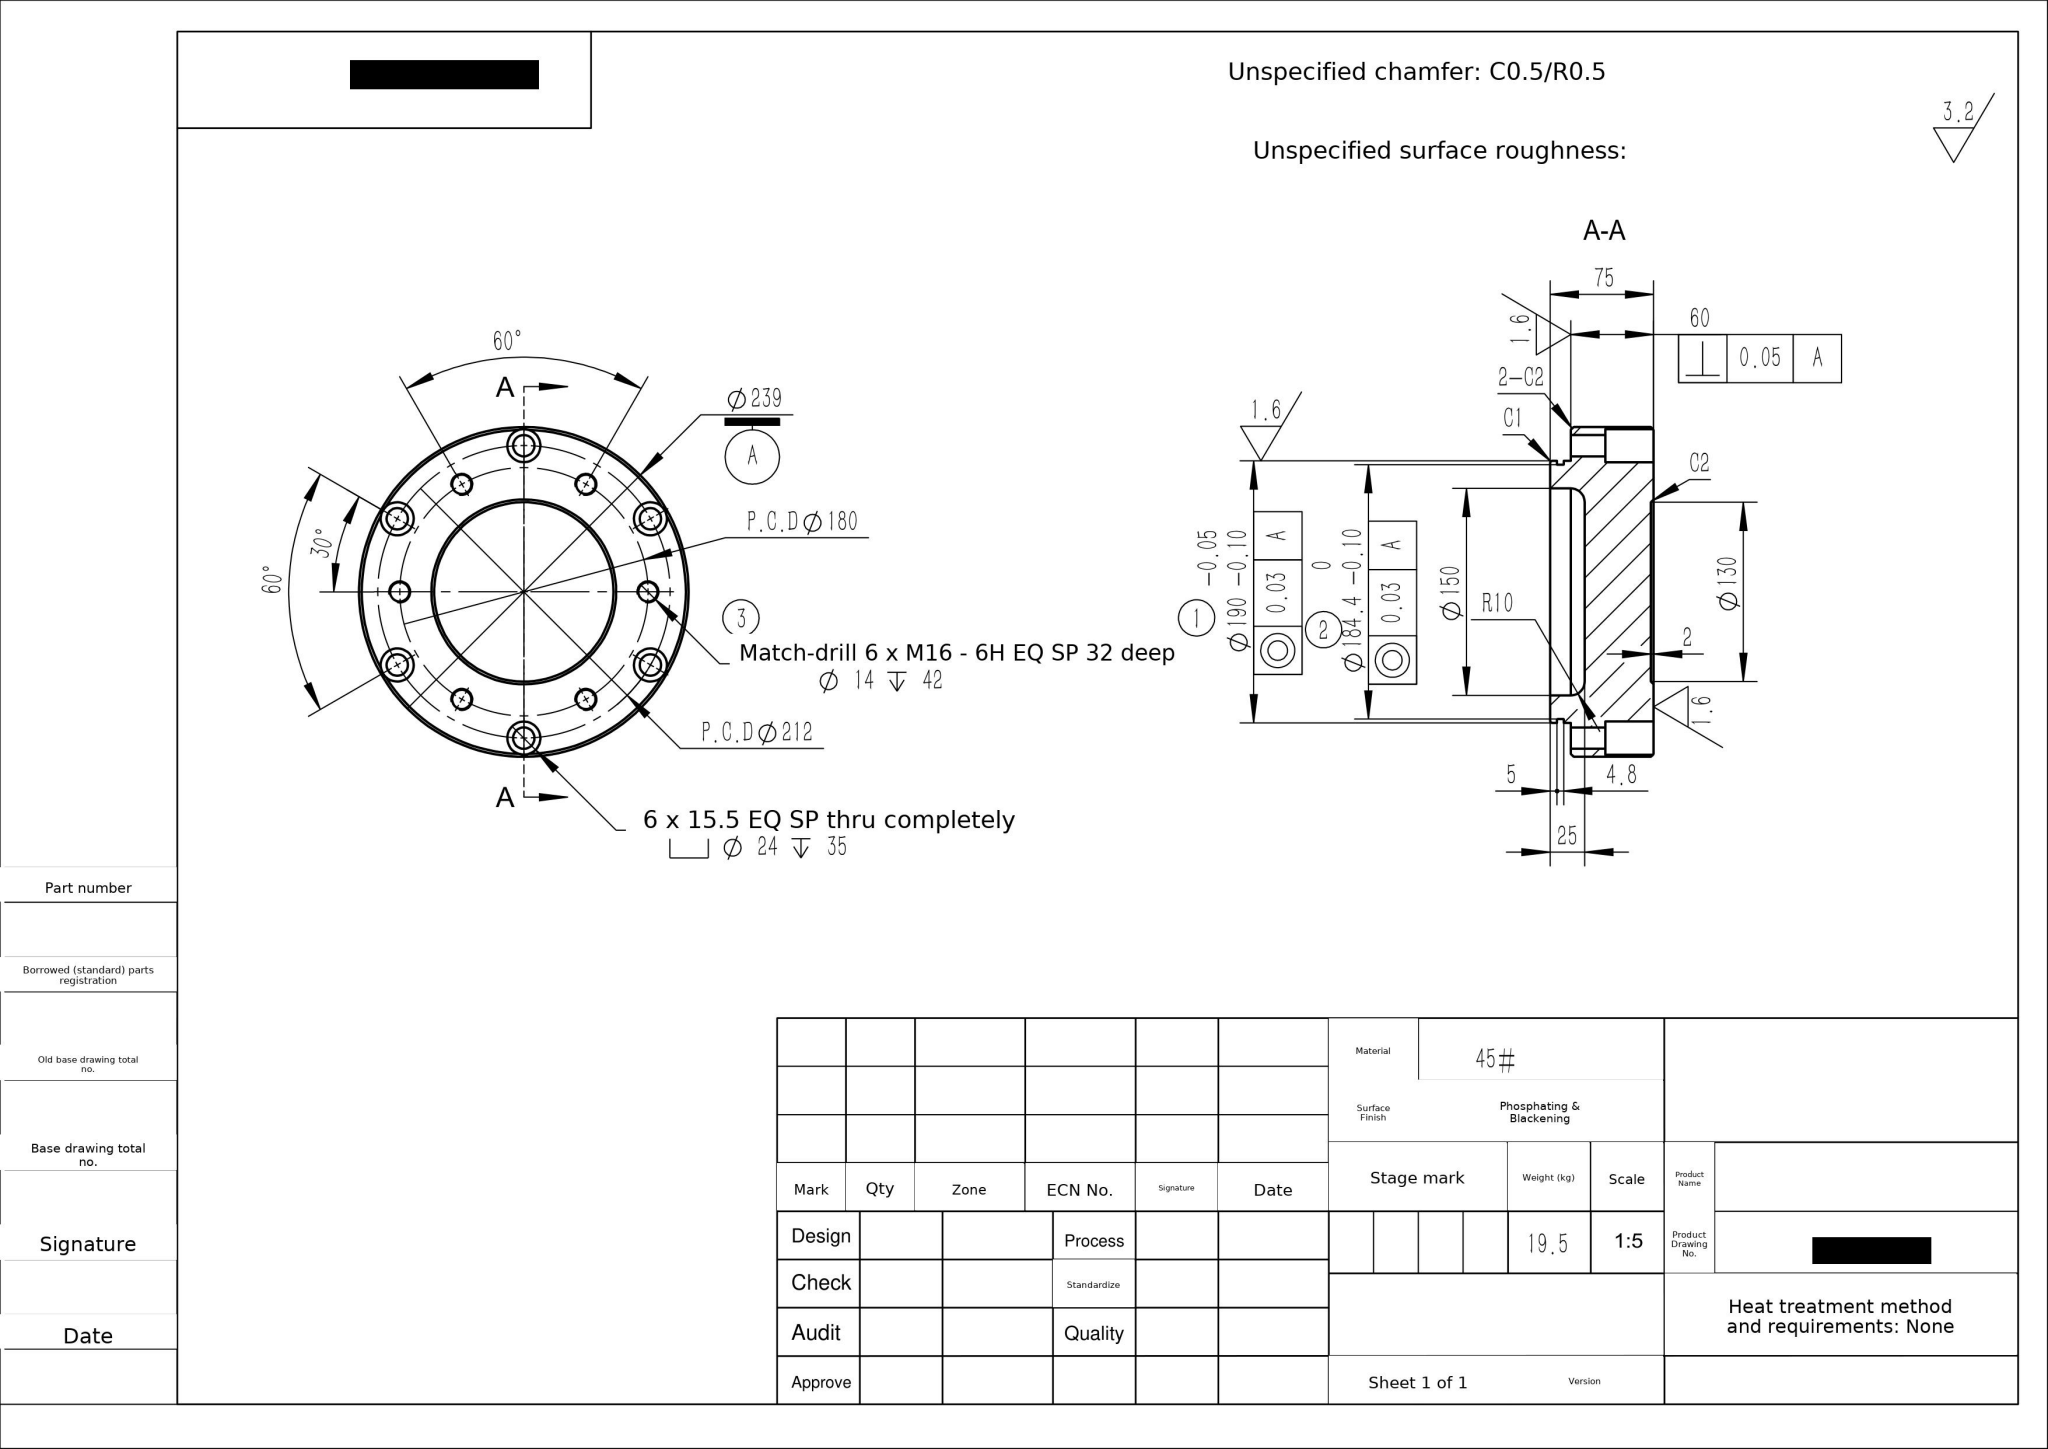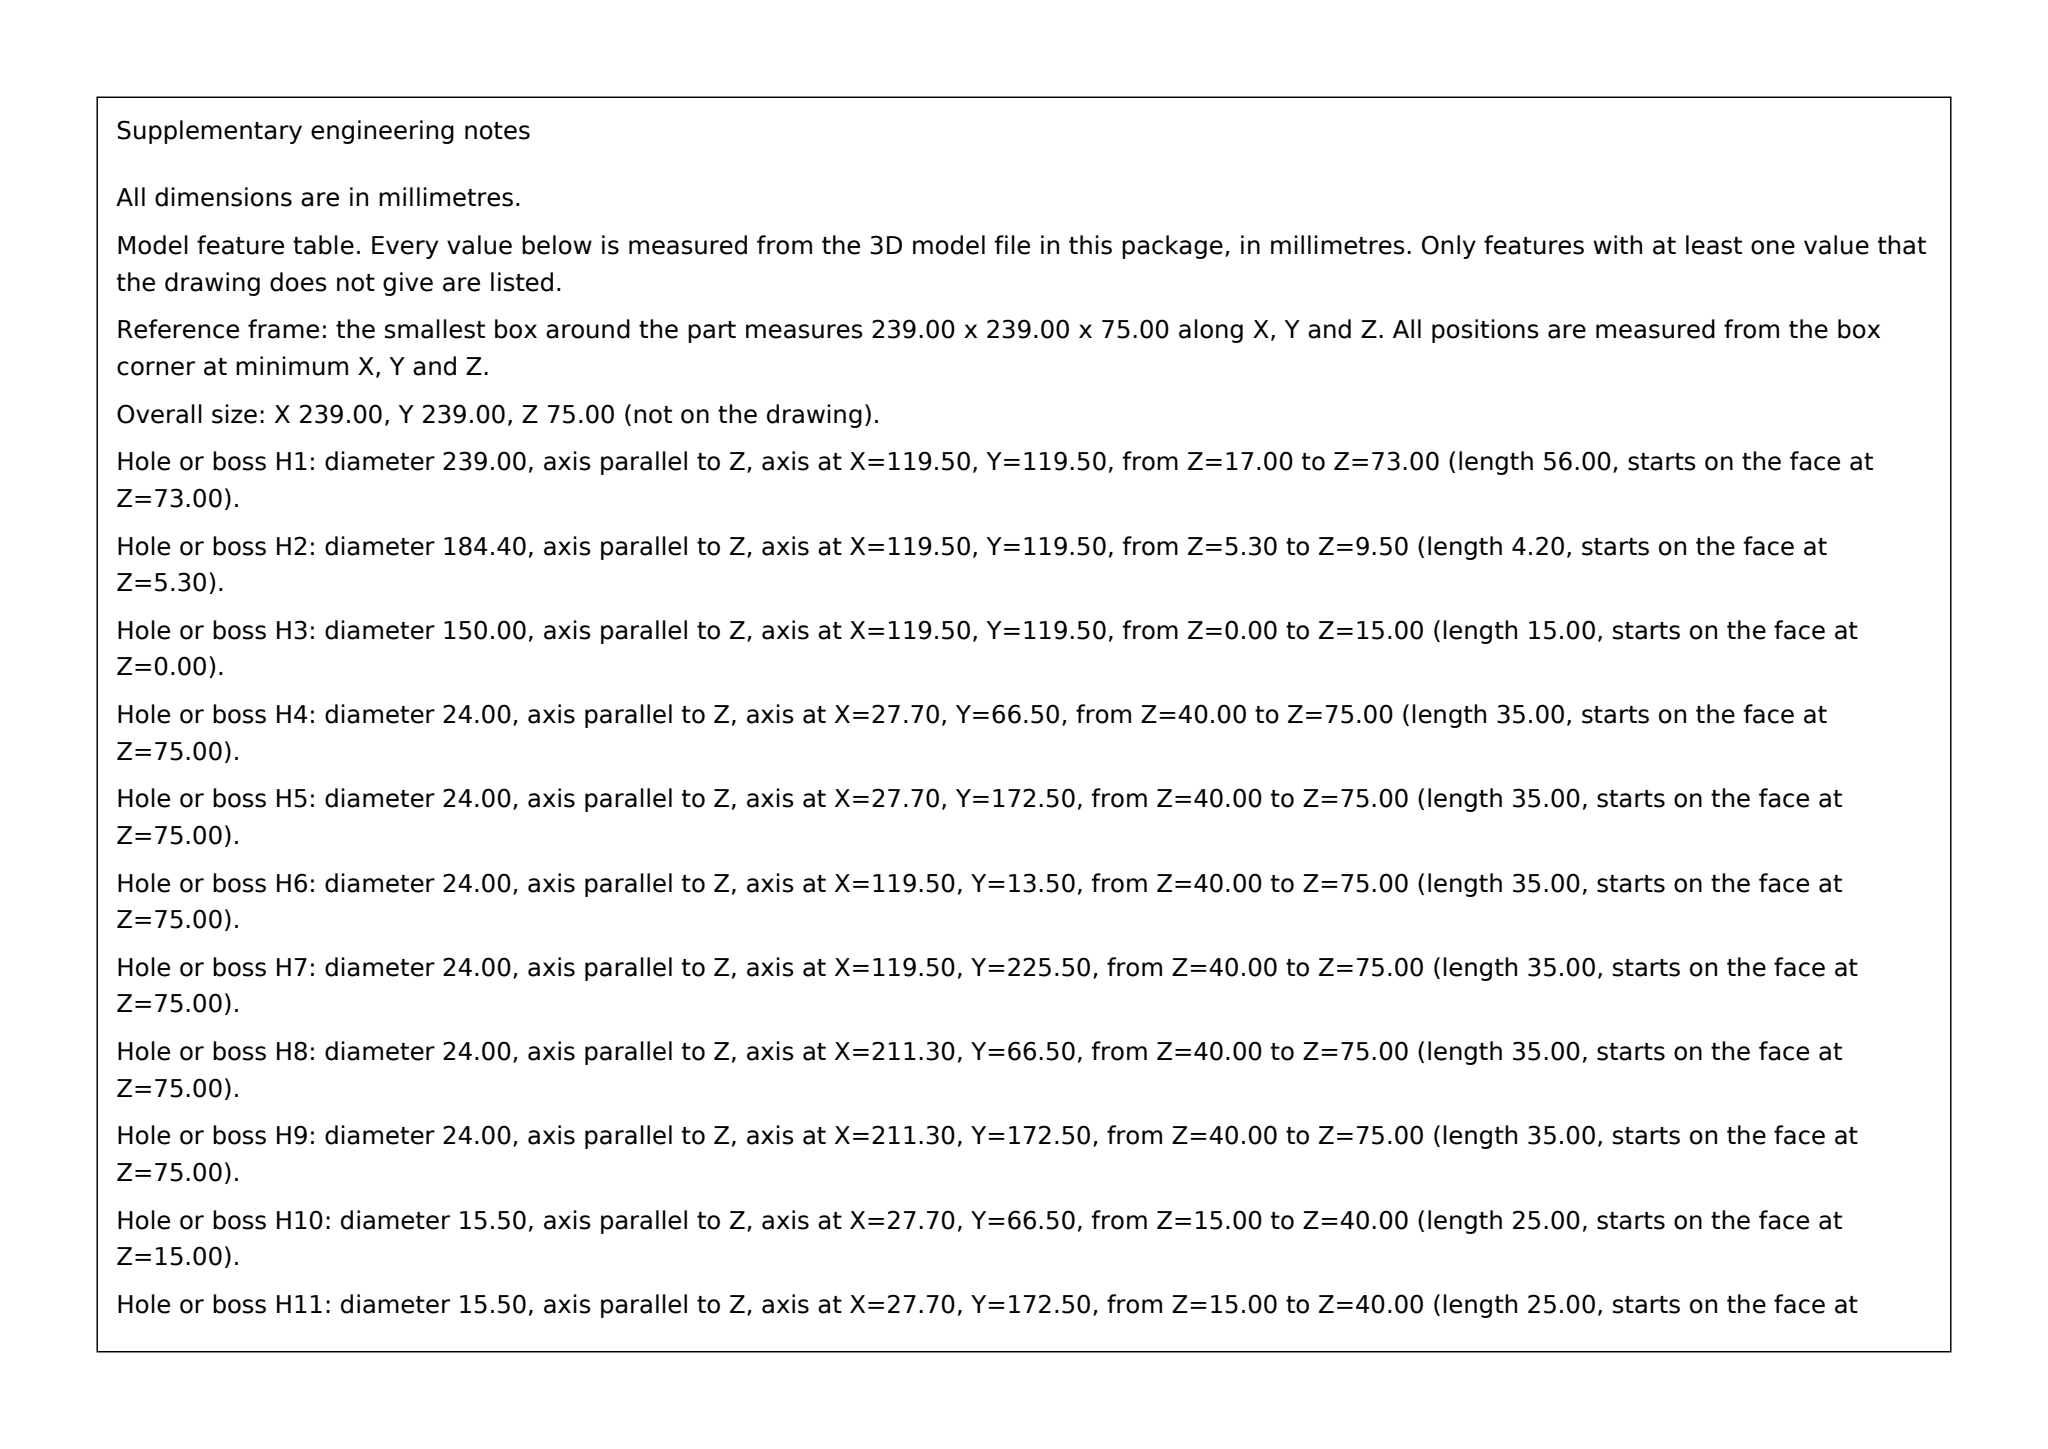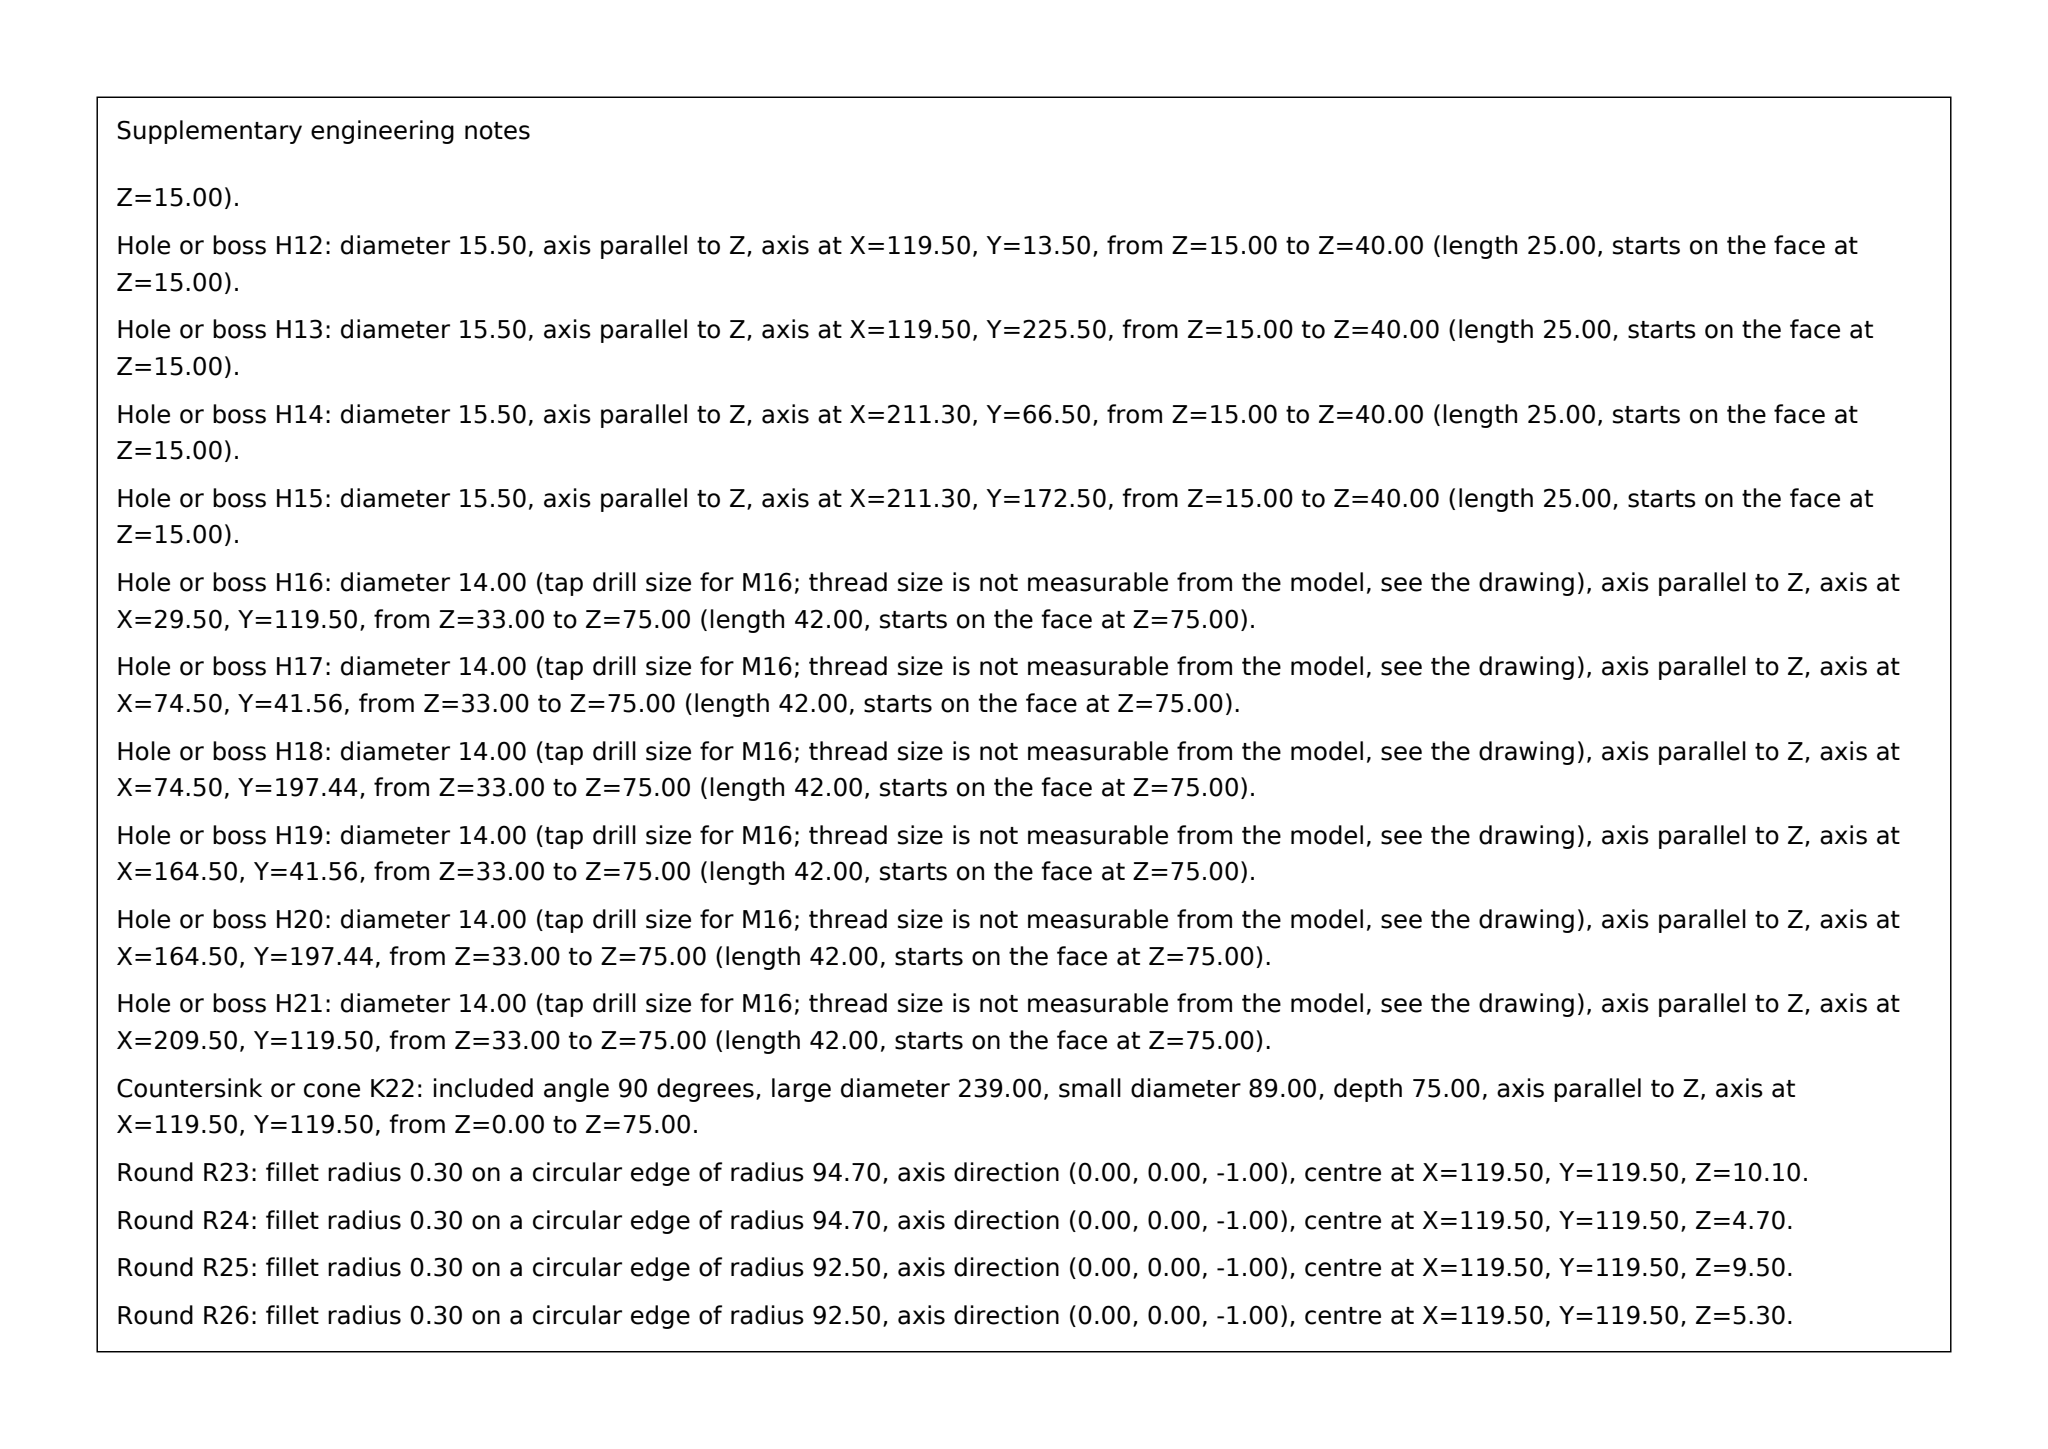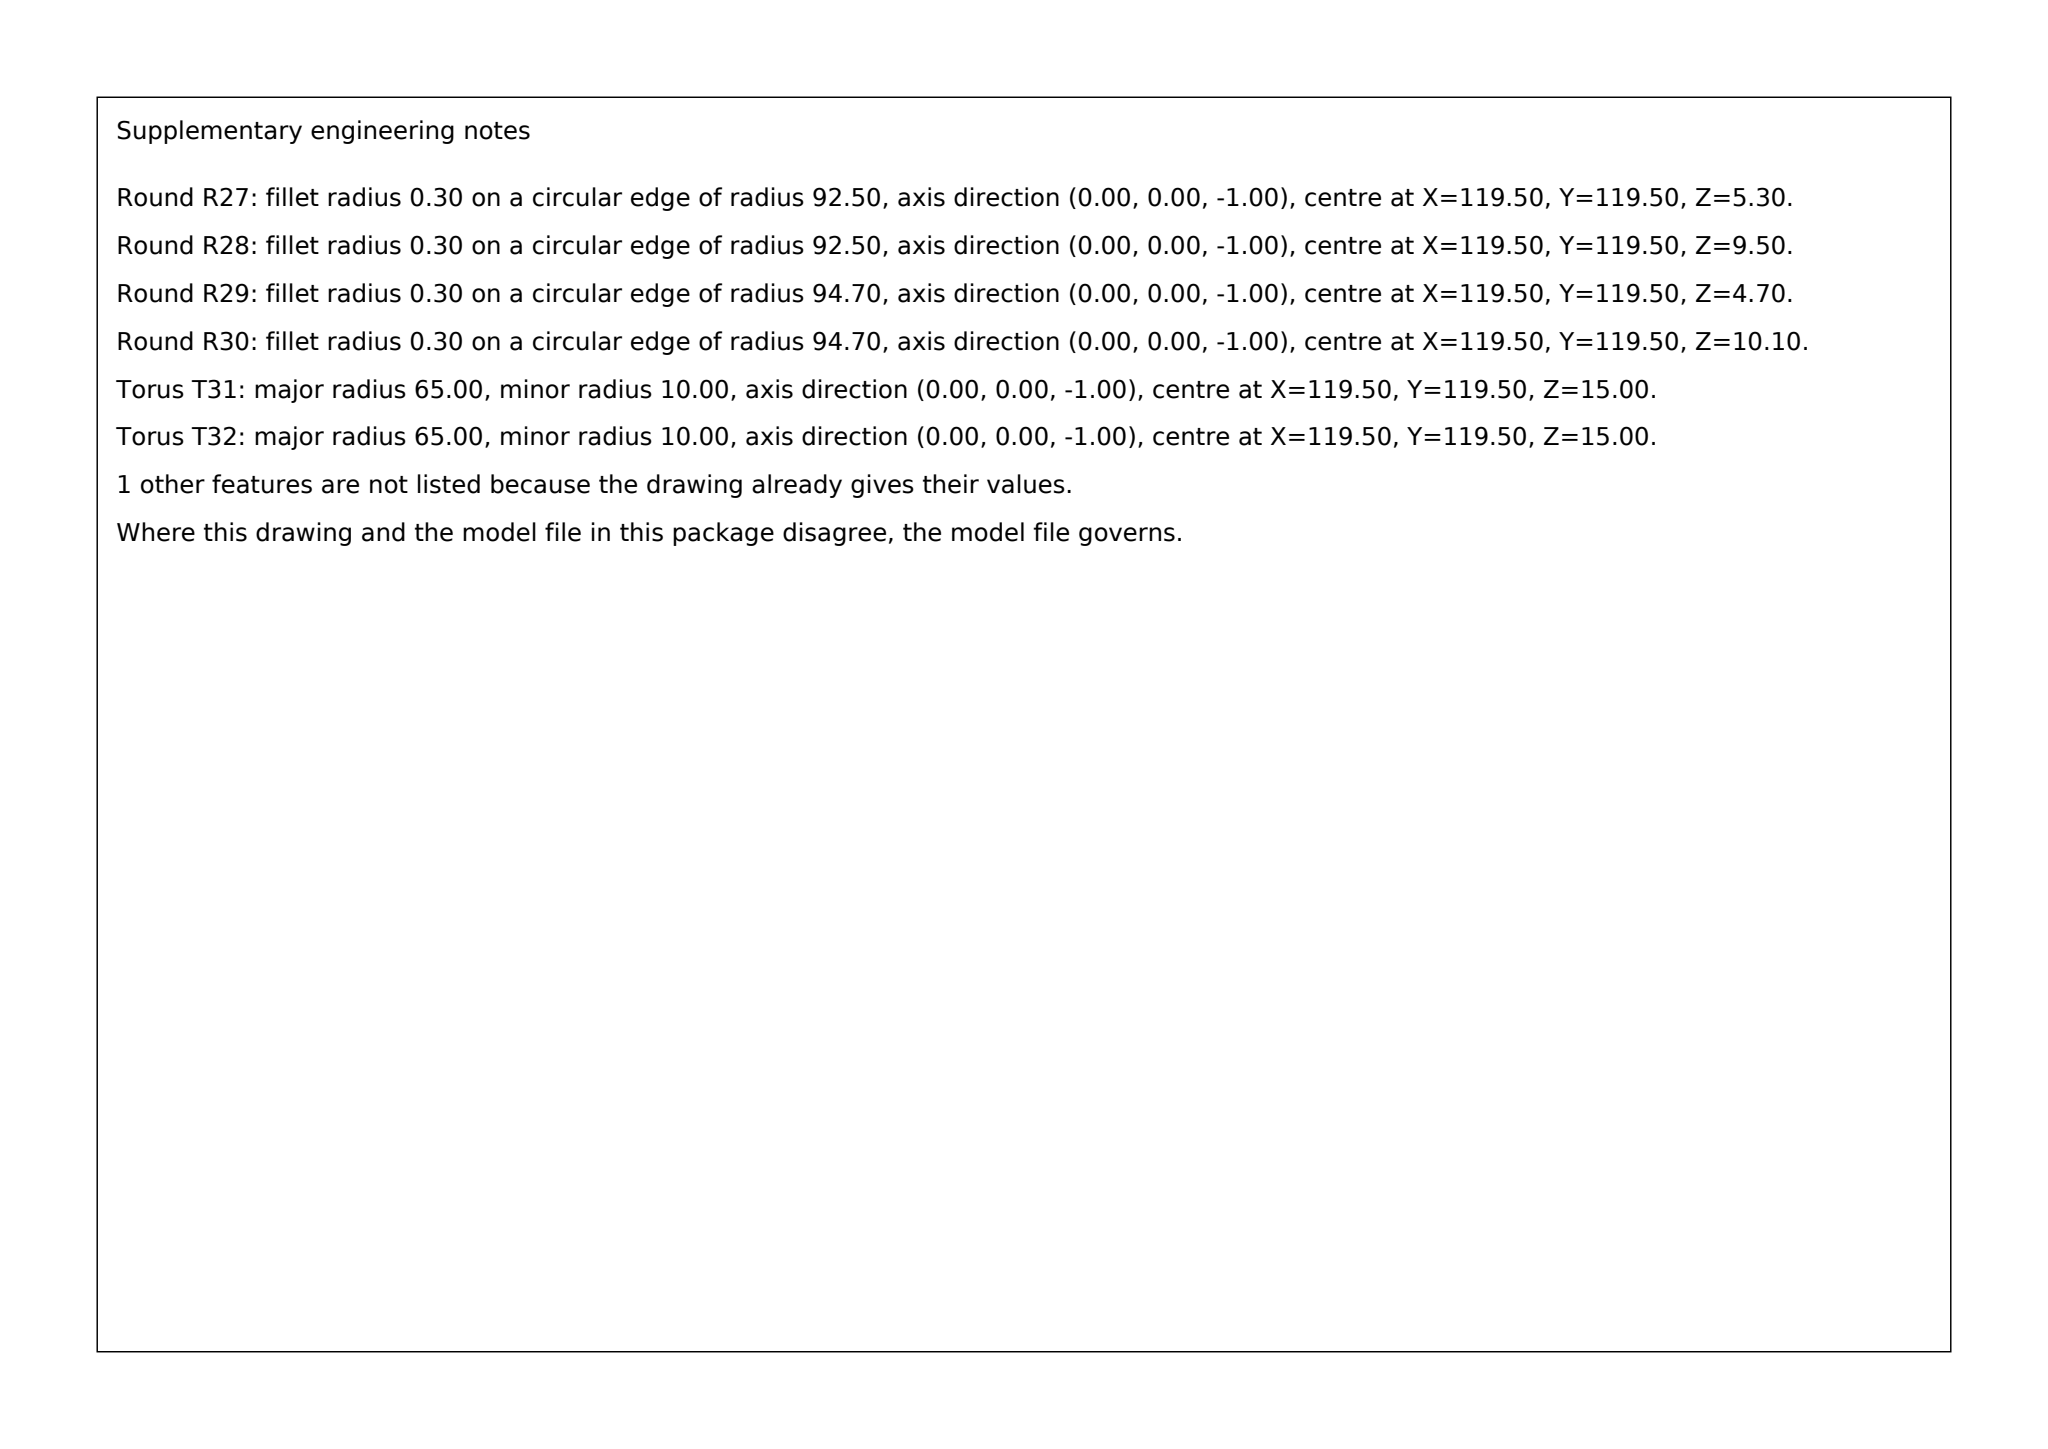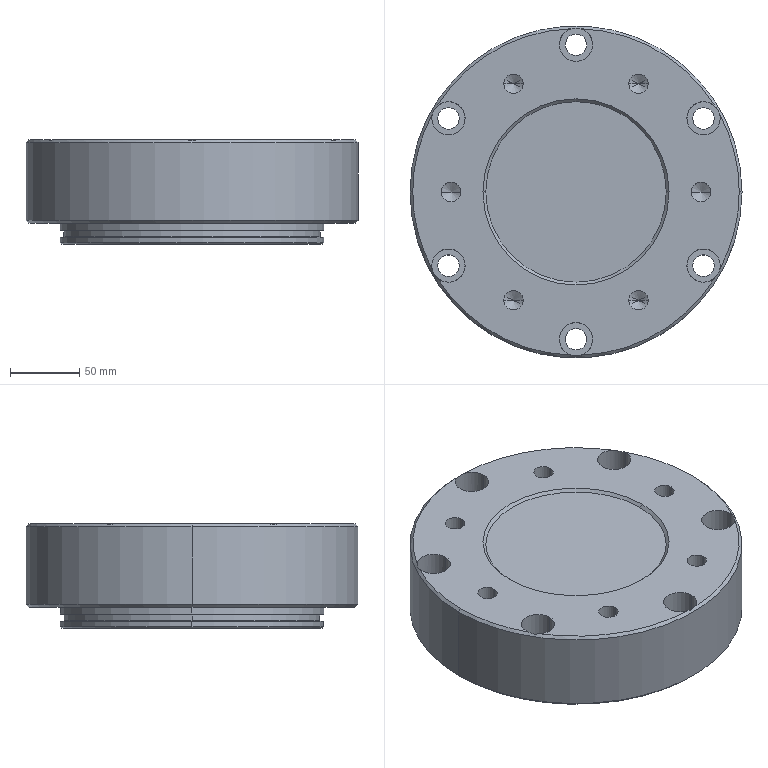Part | SolidWorks | mm | material 45# | 1 solid | 89 faces | box 239 x 239 x 75 mm | volume 2483132 mm3 | cylinder 46 | cone 20 | plane 13 | torus 10 | commonest cylinder face diameters 24 x12 15.5 x12 14 x12 190 x4 150 x2 184.4 x2 239 x2